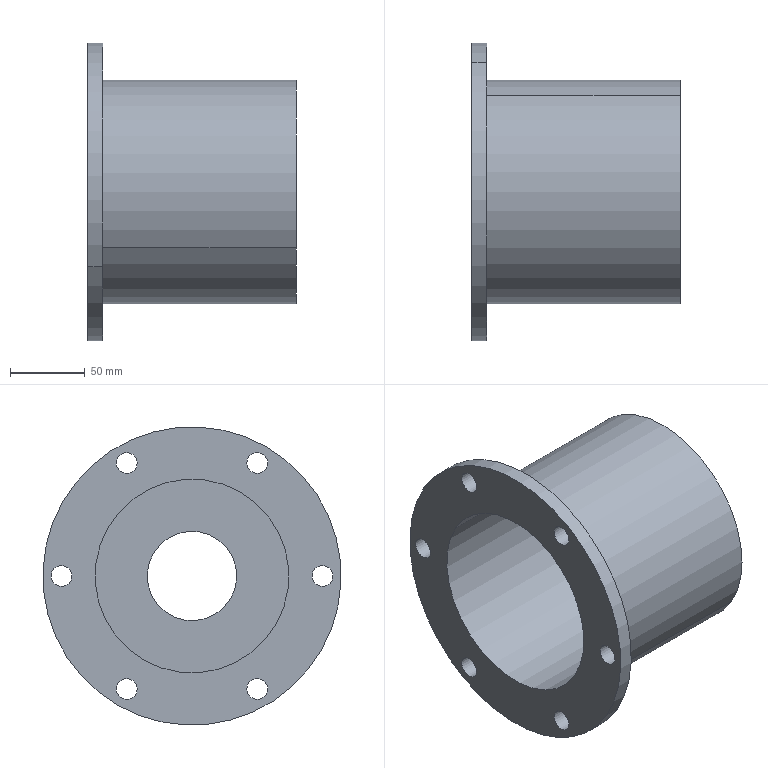Component | SolidWorks | CouplerMountingPlate-2 | 1 solid | 24 faces | box 140 x 200 x 200 mm | volume 827527 mm3 | cylinder 20 | plane 4 | commonest cylinder face diameters 14 x12 60 x2 130 x2 150 x2 200 x2
build123d program:
from build123d import *

# Parameters (mm, degrees)
SKETCH1_R           = 100
BOSS_EXTRUDE1_DEPTH = 10
SKETCH2_R           = 7
CUT_EXTRUDE1_DEPTH  = 10
CIRPATTERN1_COUNT   = 6
SKETCH3_R           = 75
BOSS_EXTRUDE2_DEPTH = 130
SKETCH4_R           = 65
CUT_EXTRUDE2_DEPTH  = 132
CUT_EXTRUDE3_REACH  = 200.997
SKETCH5_R           = 30


with BuildPart() as part:
    # Sketch1 → Boss-Extrude1 (new body)
    with BuildSketch(Plane.XY):
        Circle(SKETCH1_R)
    extrude(amount=BOSS_EXTRUDE1_DEPTH)

    # Sketch2 → Cut-Extrude1 (cut)
    with BuildSketch(Plane.XY.offset(10)):
        with Locations((0, 87.5)):
            Circle(SKETCH2_R)
    cut_extrude1 = extrude(amount=-CUT_EXTRUDE1_DEPTH, mode=Mode.SUBTRACT)

    # CirPattern1: Cut-Extrude1 ×6 about axis
    cirpattern1_axis = Axis((0, 0, 0), (0, 0, 1))
    for i in range(1, CIRPATTERN1_COUNT):
        add(cut_extrude1.rotate(cirpattern1_axis, i * 360 / CIRPATTERN1_COUNT), mode=Mode.SUBTRACT)

    # Sketch3 → Boss-Extrude2 (add)
    with BuildSketch(Plane.XY.offset(10)):
        Circle(SKETCH3_R)
    extrude(amount=BOSS_EXTRUDE2_DEPTH)

    # Sketch4 → Cut-Extrude2 (cut)
    with BuildSketch(Plane(origin=(0, 0, 0), x_dir=(-1, 0, 0), z_dir=(0, 0, -1))):
        Circle(SKETCH4_R)
    extrude(amount=-CUT_EXTRUDE2_DEPTH, mode=Mode.SUBTRACT)

    # Sketch5 → Cut-Extrude3 (cut, up to next)
    with BuildSketch(Plane.XY.offset(140), mode=Mode.PRIVATE) as cut_extrude3_sk1:
        Circle(SKETCH5_R)
    cut_extrude3_tool1 = extrude(cut_extrude3_sk1.sketch, amount=-CUT_EXTRUDE3_REACH, mode=Mode.PRIVATE) & part.part
    add(cut_extrude3_tool1.solids().sort_by_distance((0, 0, 140))[0], mode=Mode.SUBTRACT)


solid = part.part

# Placed as in the assembly
solid = solid.moved(Location((115.641, 70.663, 0), (0, 90, 0)))